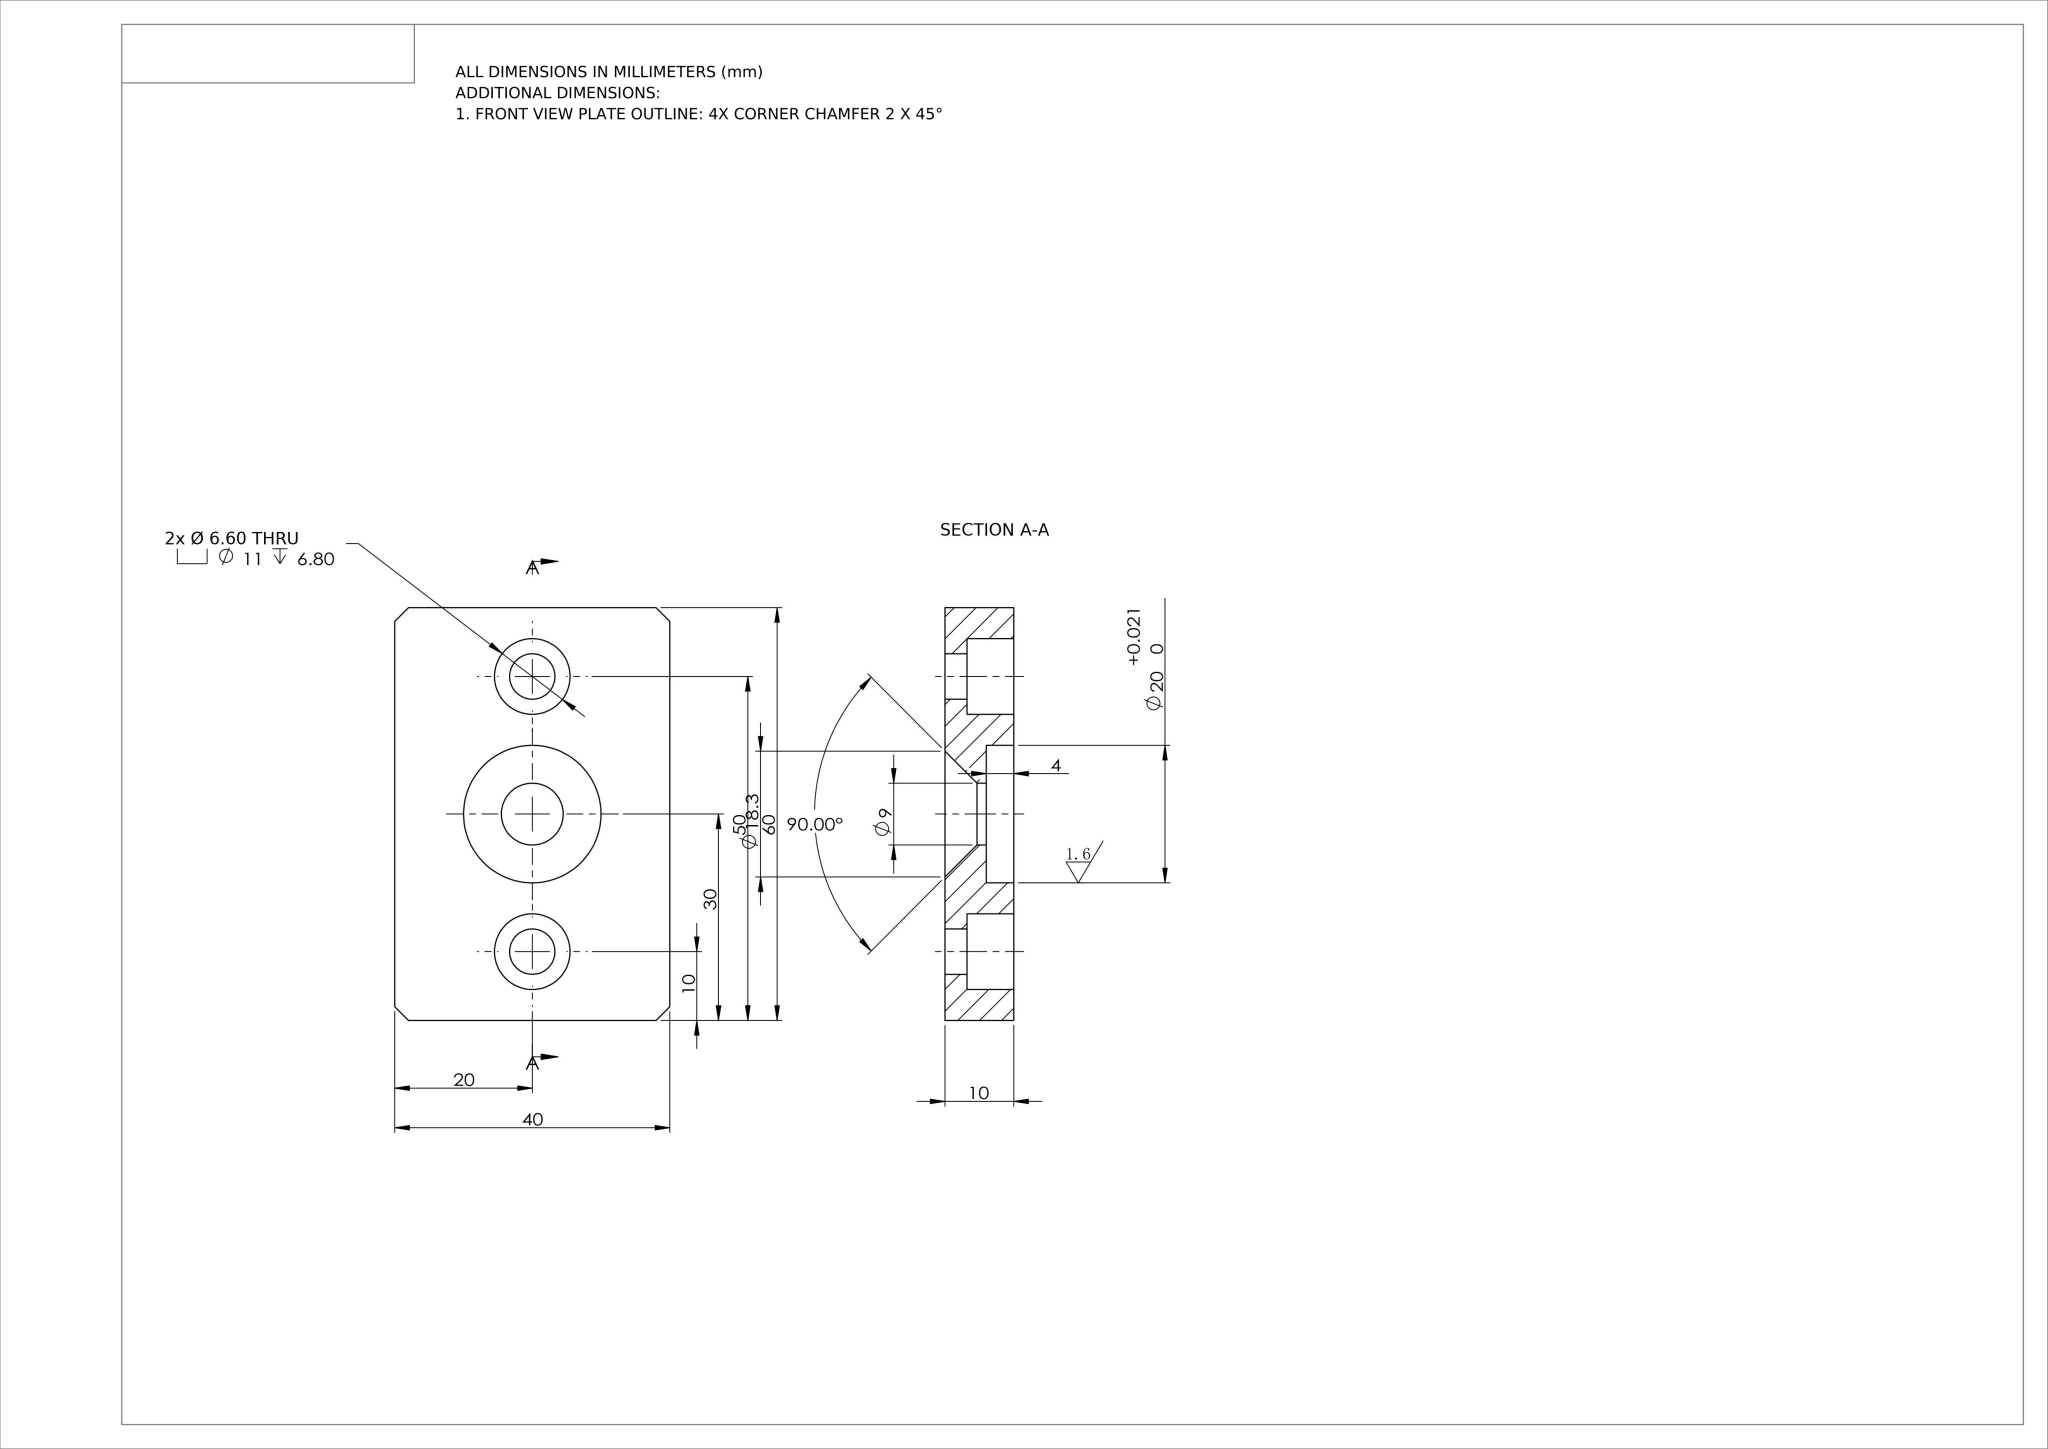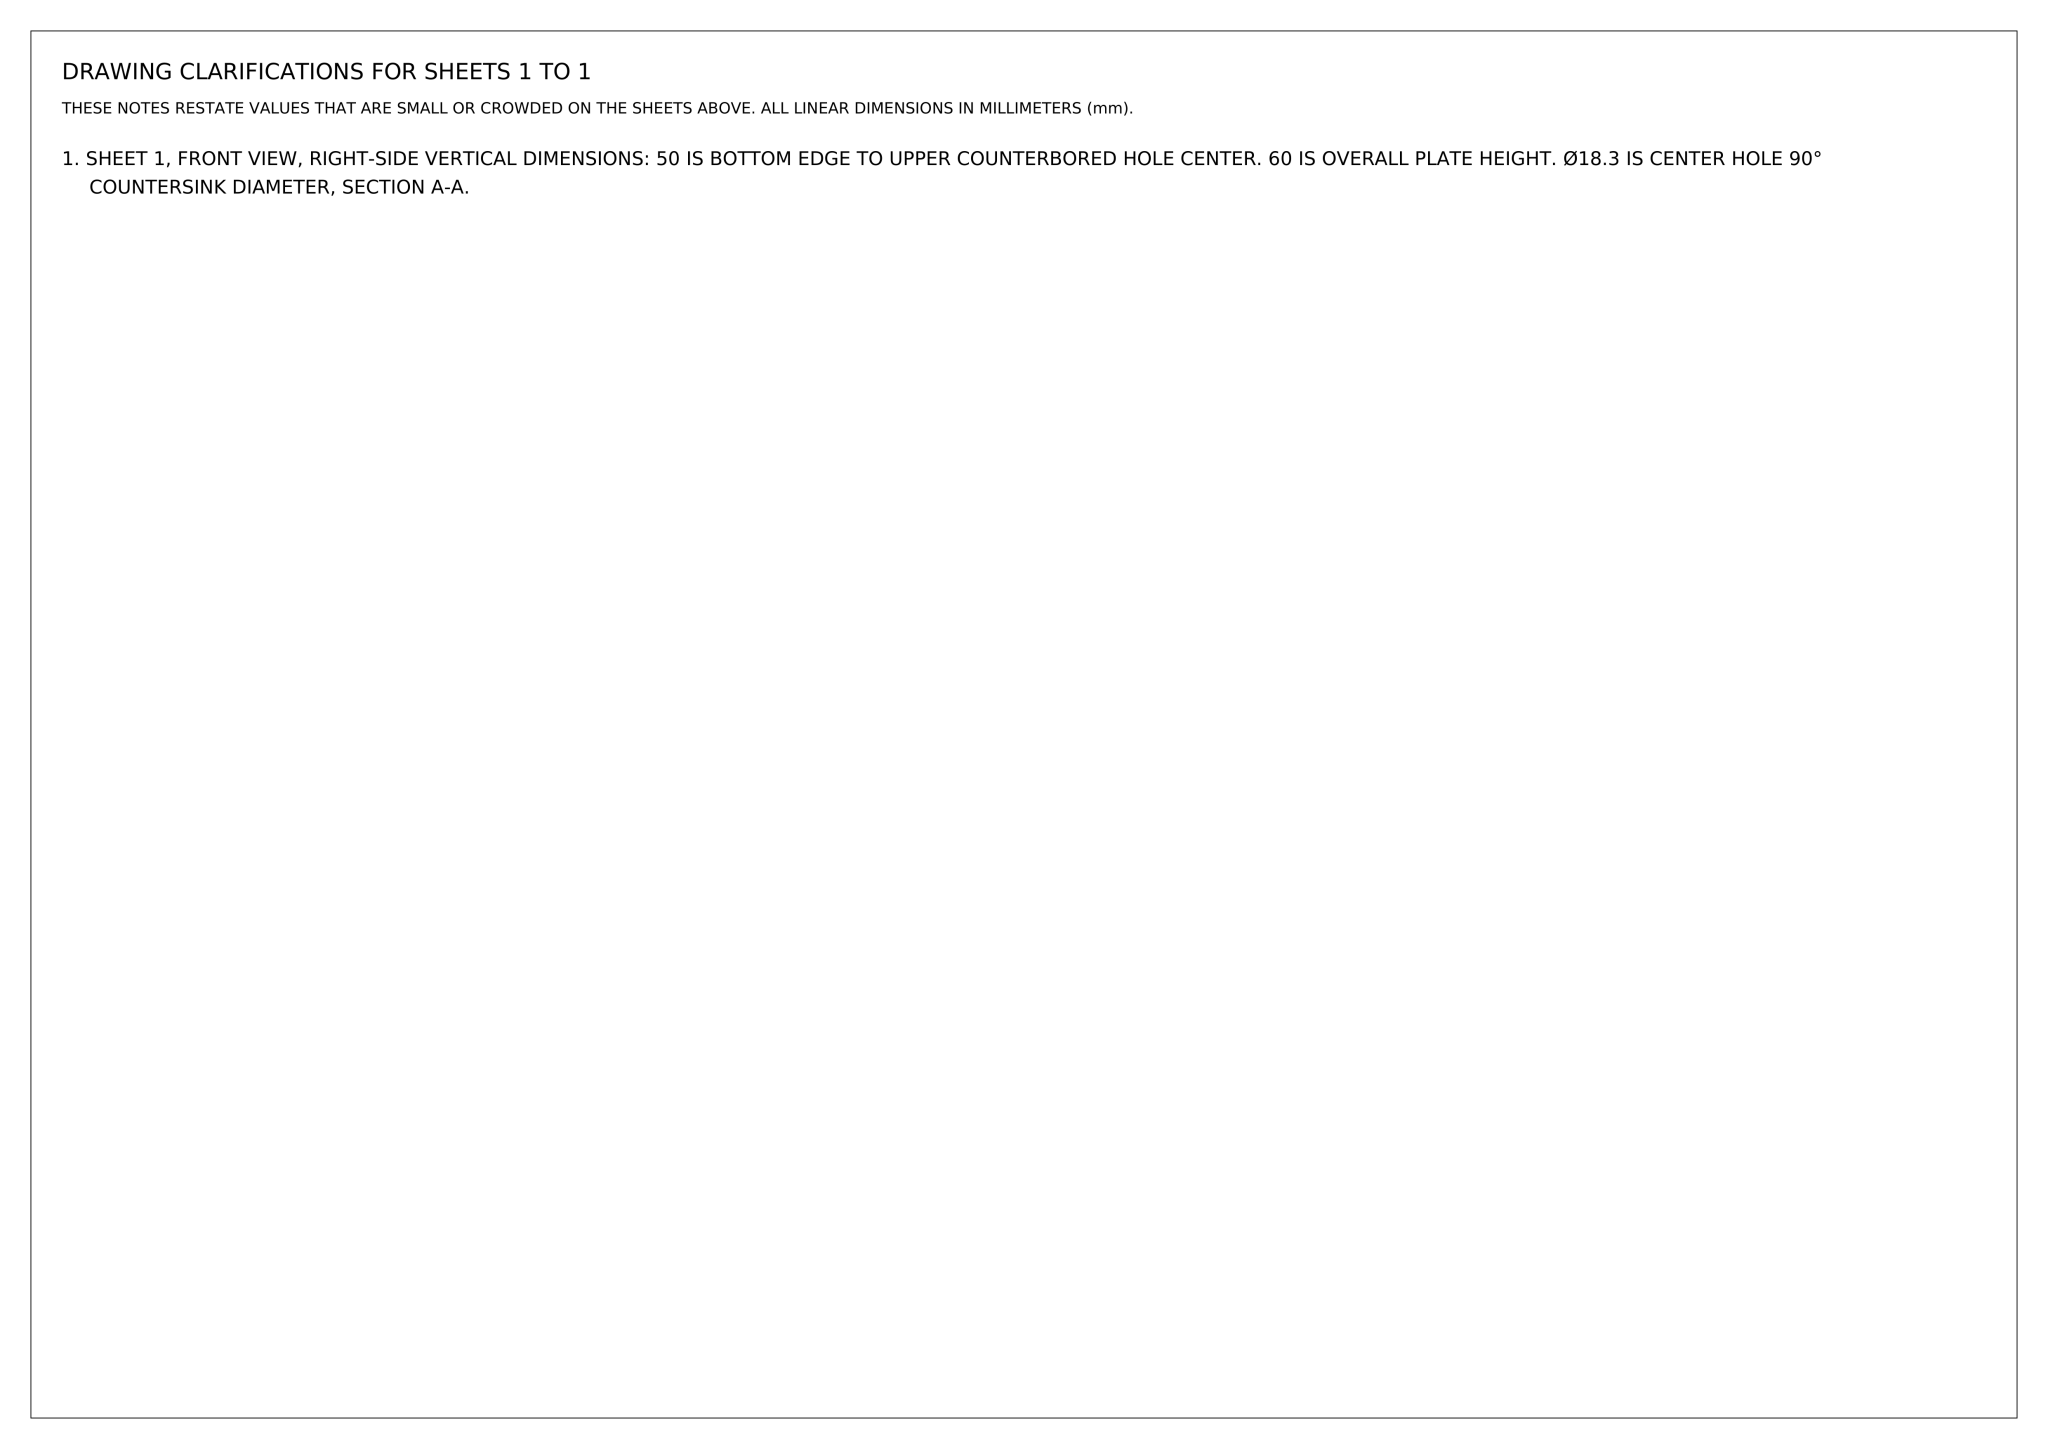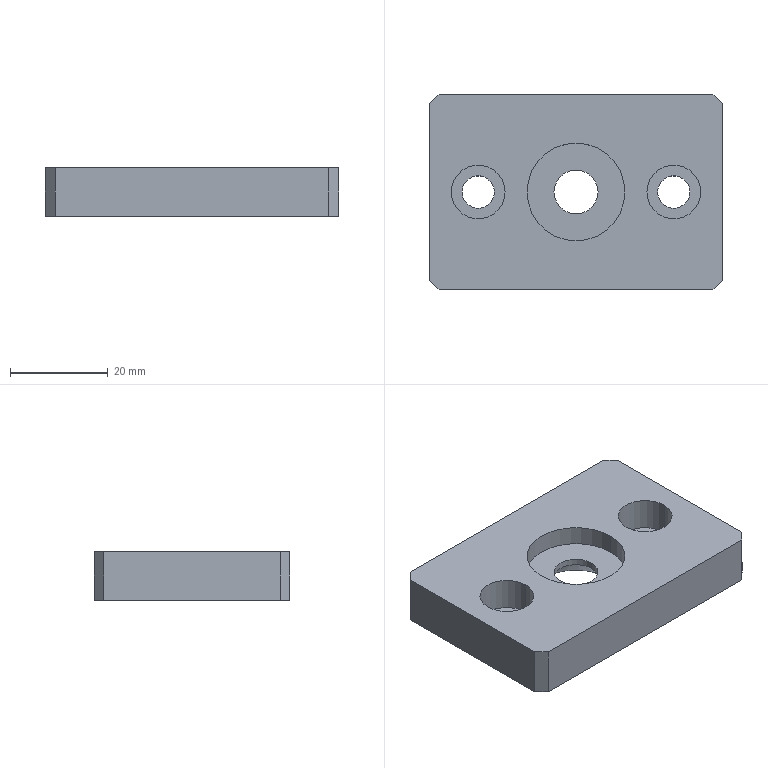Part | NX | mm | 1 solid | 27 faces | box 60 x 40 x 10 mm | volume 20359 mm3 | plane 13 | cylinder 12 | cone 2 | commonest cylinder face diameters 11 x4 6.6 x4 9 x2 20 x2
STEP:
#1=COLOUR_RGB('',0.6157,0.6431,0.6745);
#2=FILL_AREA_STYLE_COLOUR('',#1);
#3=FILL_AREA_STYLE('',(#2));
#4=SURFACE_STYLE_FILL_AREA(#3);
#5=SURFACE_SIDE_STYLE('',(#4));
#6=SURFACE_STYLE_USAGE(.BOTH.,#5);
#7=PRESENTATION_STYLE_ASSIGNMENT((#6));
#8=CARTESIAN_POINT('',(-25.5,-0.,3.2));
#9=VERTEX_POINT('',#8);
#10=CARTESIAN_POINT('',(-14.5,-0.,3.2));
#11=VERTEX_POINT('',#10);
#12=CARTESIAN_POINT('',(-20.,-0.,3.2));
#13=DIRECTION('',(0.,0.,1.));
#14=DIRECTION('',(1.,0.,0.));
#15=AXIS2_PLACEMENT_3D('',#12,#13,#14);
#16=CIRCLE('',#15,5.5);
#17=EDGE_CURVE('',#9,#11,#16,.T.);
#18=ORIENTED_EDGE('',*,*,#17,.F.);
#19=CARTESIAN_POINT('',(-25.5,-0.,10.));
#20=VERTEX_POINT('',#19);
#21=CARTESIAN_POINT('',(-25.5,-0.,10.));
#22=DIRECTION('',(0.,0.,1.));
#23=VECTOR('',#22,1000.);
#24=LINE('',#21,#23);
#25=EDGE_CURVE('',#9,#20,#24,.T.);
#26=ORIENTED_EDGE('',*,*,#25,.T.);
#27=CARTESIAN_POINT('',(-14.5,-0.,10.));
#28=VERTEX_POINT('',#27);
#29=CARTESIAN_POINT('',(-20.,-0.,10.));
#30=DIRECTION('',(0.,0.,1.));
#31=DIRECTION('',(1.,0.,0.));
#32=AXIS2_PLACEMENT_3D('',#29,#30,#31);
#33=CIRCLE('',#32,5.5);
#34=EDGE_CURVE('',#20,#28,#33,.T.);
#35=ORIENTED_EDGE('',*,*,#34,.T.);
#36=CARTESIAN_POINT('',(-14.5,-0.,10.));
#37=DIRECTION('',(0.,0.,1.));
#38=VECTOR('',#37,1000.);
#39=LINE('',#36,#38);
#40=EDGE_CURVE('',#11,#28,#39,.T.);
#41=ORIENTED_EDGE('',*,*,#40,.F.);
#42=EDGE_LOOP('',(#18,#26,#35,#41));
#43=FACE_OUTER_BOUND('',#42,.T.);
#44=CARTESIAN_POINT('',(-20.,-0.,10.));
#45=DIRECTION('',(0.,0.,1.));
#46=DIRECTION('',(1.,0.,0.));
#47=AXIS2_PLACEMENT_3D('',#44,#45,#46);
#48=CYLINDRICAL_SURFACE('',#47,5.5);
#49=ADVANCED_FACE('',(#43),#48,.F.);
#50=CARTESIAN_POINT('',(-23.3,-0.,0.));
#51=VERTEX_POINT('',#50);
#52=CARTESIAN_POINT('',(-16.7,-0.,0.));
#53=VERTEX_POINT('',#52);
#54=CARTESIAN_POINT('',(-20.,-0.,0.));
#55=DIRECTION('',(0.,0.,1.));
#56=DIRECTION('',(1.,0.,0.));
#57=AXIS2_PLACEMENT_3D('',#54,#55,#56);
#58=CIRCLE('',#57,3.3);
#59=EDGE_CURVE('',#51,#53,#58,.T.);
#60=ORIENTED_EDGE('',*,*,#59,.F.);
#61=CARTESIAN_POINT('',(-23.3,-0.,3.2));
#62=VERTEX_POINT('',#61);
#63=CARTESIAN_POINT('',(-23.3,-0.,10.));
#64=DIRECTION('',(0.,0.,1.));
#65=VECTOR('',#64,1000.);
#66=LINE('',#63,#65);
#67=EDGE_CURVE('',#51,#62,#66,.T.);
#68=ORIENTED_EDGE('',*,*,#67,.T.);
#69=CARTESIAN_POINT('',(-16.7,-0.,3.2));
#70=VERTEX_POINT('',#69);
#71=CARTESIAN_POINT('',(-20.,-0.,3.2));
#72=DIRECTION('',(0.,0.,1.));
#73=DIRECTION('',(1.,0.,0.));
#74=AXIS2_PLACEMENT_3D('',#71,#72,#73);
#75=CIRCLE('',#74,3.3);
#76=EDGE_CURVE('',#62,#70,#75,.T.);
#77=ORIENTED_EDGE('',*,*,#76,.T.);
#78=CARTESIAN_POINT('',(-16.7,-0.,10.));
#79=DIRECTION('',(0.,0.,1.));
#80=VECTOR('',#79,1000.);
#81=LINE('',#78,#80);
#82=EDGE_CURVE('',#53,#70,#81,.T.);
#83=ORIENTED_EDGE('',*,*,#82,.F.);
#84=EDGE_LOOP('',(#60,#68,#77,#83));
#85=FACE_OUTER_BOUND('',#84,.T.);
#86=CARTESIAN_POINT('',(-20.,-0.,10.));
#87=DIRECTION('',(0.,0.,1.));
#88=DIRECTION('',(1.,0.,0.));
#89=AXIS2_PLACEMENT_3D('',#86,#87,#88);
#90=CYLINDRICAL_SURFACE('',#89,3.3);
#91=ADVANCED_FACE('',(#85),#90,.F.);
#92=CARTESIAN_POINT('',(14.5,0.,3.2));
#93=VERTEX_POINT('',#92);
#94=CARTESIAN_POINT('',(25.5,0.,3.2));
#95=VERTEX_POINT('',#94);
#96=CARTESIAN_POINT('',(20.,0.,3.2));
#97=DIRECTION('',(0.,0.,1.));
#98=DIRECTION('',(1.,0.,0.));
#99=AXIS2_PLACEMENT_3D('',#96,#97,#98);
#100=CIRCLE('',#99,5.5);
#101=EDGE_CURVE('',#93,#95,#100,.T.);
#102=ORIENTED_EDGE('',*,*,#101,.F.);
#103=CARTESIAN_POINT('',(14.5,0.,10.));
#104=VERTEX_POINT('',#103);
#105=CARTESIAN_POINT('',(14.5,0.,10.));
#106=DIRECTION('',(0.,0.,1.));
#107=VECTOR('',#106,1000.);
#108=LINE('',#105,#107);
#109=EDGE_CURVE('',#93,#104,#108,.T.);
#110=ORIENTED_EDGE('',*,*,#109,.T.);
#111=CARTESIAN_POINT('',(25.5,0.,10.));
#112=VERTEX_POINT('',#111);
#113=CARTESIAN_POINT('',(20.,0.,10.));
#114=DIRECTION('',(0.,0.,1.));
#115=DIRECTION('',(1.,0.,0.));
#116=AXIS2_PLACEMENT_3D('',#113,#114,#115);
#117=CIRCLE('',#116,5.5);
#118=EDGE_CURVE('',#104,#112,#117,.T.);
#119=ORIENTED_EDGE('',*,*,#118,.T.);
#120=CARTESIAN_POINT('',(25.5,0.,10.));
#121=DIRECTION('',(0.,0.,1.));
#122=VECTOR('',#121,1000.);
#123=LINE('',#120,#122);
#124=EDGE_CURVE('',#95,#112,#123,.T.);
#125=ORIENTED_EDGE('',*,*,#124,.F.);
#126=EDGE_LOOP('',(#102,#110,#119,#125));
#127=FACE_OUTER_BOUND('',#126,.T.);
#128=CARTESIAN_POINT('',(20.,0.,10.));
#129=DIRECTION('',(0.,0.,1.));
#130=DIRECTION('',(1.,0.,0.));
#131=AXIS2_PLACEMENT_3D('',#128,#129,#130);
#132=CYLINDRICAL_SURFACE('',#131,5.5);
#133=ADVANCED_FACE('',(#127),#132,.F.);
#134=CARTESIAN_POINT('',(16.7,0.,0.));
#135=VERTEX_POINT('',#134);
#136=CARTESIAN_POINT('',(23.3,0.,0.));
#137=VERTEX_POINT('',#136);
#138=CARTESIAN_POINT('',(20.,0.,0.));
#139=DIRECTION('',(0.,0.,1.));
#140=DIRECTION('',(1.,0.,0.));
#141=AXIS2_PLACEMENT_3D('',#138,#139,#140);
#142=CIRCLE('',#141,3.3);
#143=EDGE_CURVE('',#135,#137,#142,.T.);
#144=ORIENTED_EDGE('',*,*,#143,.F.);
#145=CARTESIAN_POINT('',(16.7,0.,3.2));
#146=VERTEX_POINT('',#145);
#147=CARTESIAN_POINT('',(16.7,0.,10.));
#148=DIRECTION('',(0.,0.,1.));
#149=VECTOR('',#148,1000.);
#150=LINE('',#147,#149);
#151=EDGE_CURVE('',#135,#146,#150,.T.);
#152=ORIENTED_EDGE('',*,*,#151,.T.);
#153=CARTESIAN_POINT('',(23.3,0.,3.2));
#154=VERTEX_POINT('',#153);
#155=CARTESIAN_POINT('',(20.,0.,3.2));
#156=DIRECTION('',(0.,0.,1.));
#157=DIRECTION('',(1.,0.,0.));
#158=AXIS2_PLACEMENT_3D('',#155,#156,#157);
#159=CIRCLE('',#158,3.3);
#160=EDGE_CURVE('',#146,#154,#159,.T.);
#161=ORIENTED_EDGE('',*,*,#160,.T.);
#162=CARTESIAN_POINT('',(23.3,0.,10.));
#163=DIRECTION('',(0.,0.,1.));
#164=VECTOR('',#163,1000.);
#165=LINE('',#162,#164);
#166=EDGE_CURVE('',#137,#154,#165,.T.);
#167=ORIENTED_EDGE('',*,*,#166,.F.);
#168=EDGE_LOOP('',(#144,#152,#161,#167));
#169=FACE_OUTER_BOUND('',#168,.T.);
#170=CARTESIAN_POINT('',(20.,0.,10.));
#171=DIRECTION('',(0.,0.,1.));
#172=DIRECTION('',(1.,0.,0.));
#173=AXIS2_PLACEMENT_3D('',#170,#171,#172);
#174=CYLINDRICAL_SURFACE('',#173,3.3);
#175=ADVANCED_FACE('',(#169),#174,.F.);
#176=CARTESIAN_POINT('',(4.5,0.,4.65));
#177=VERTEX_POINT('',#176);
#178=CARTESIAN_POINT('',(-4.5,-0.,4.65));
#179=VERTEX_POINT('',#178);
#180=CARTESIAN_POINT('',(0.,0.,4.65));
#181=DIRECTION('',(-0.,-0.,-1.));
#182=DIRECTION('',(-1.,-0.,-0.));
#183=AXIS2_PLACEMENT_3D('',#180,#181,#182);
#184=CIRCLE('',#183,4.5);
#185=EDGE_CURVE('',#177,#179,#184,.T.);
#186=ORIENTED_EDGE('',*,*,#185,.F.);
#187=CARTESIAN_POINT('',(9.15,0.,-0.));
#188=VERTEX_POINT('',#187);
#189=CARTESIAN_POINT('',(9.15,0.,0.));
#190=DIRECTION('',(0.7071,0.,-0.7071));
#191=VECTOR('',#190,1000.);
#192=LINE('',#189,#191);
#193=EDGE_CURVE('',#177,#188,#192,.T.);
#194=ORIENTED_EDGE('',*,*,#193,.T.);
#195=CARTESIAN_POINT('',(-9.15,-0.,0.));
#196=VERTEX_POINT('',#195);
#197=CARTESIAN_POINT('',(0.,0.,0.));
#198=DIRECTION('',(-0.,-0.,-1.));
#199=DIRECTION('',(-1.,-0.,-0.));
#200=AXIS2_PLACEMENT_3D('',#197,#198,#199);
#201=CIRCLE('',#200,9.15);
#202=EDGE_CURVE('',#188,#196,#201,.T.);
#203=ORIENTED_EDGE('',*,*,#202,.T.);
#204=CARTESIAN_POINT('',(-9.15,-0.,-0.));
#205=DIRECTION('',(-0.7071,-0.,-0.7071));
#206=VECTOR('',#205,1000.);
#207=LINE('',#204,#206);
#208=EDGE_CURVE('',#179,#196,#207,.T.);
#209=ORIENTED_EDGE('',*,*,#208,.F.);
#210=EDGE_LOOP('',(#186,#194,#203,#209));
#211=FACE_OUTER_BOUND('',#210,.T.);
#212=CARTESIAN_POINT('',(0.,0.,0.));
#213=DIRECTION('',(-0.,-0.,-1.));
#214=DIRECTION('',(-1.,-0.,-0.));
#215=AXIS2_PLACEMENT_3D('',#212,#213,#214);
#216=CONICAL_SURFACE('',#215,9.15,0.7854);
#217=ADVANCED_FACE('',(#211),#216,.F.);
#218=CARTESIAN_POINT('',(-4.5,-0.,6.));
#219=VERTEX_POINT('',#218);
#220=CARTESIAN_POINT('',(4.5,0.,6.));
#221=VERTEX_POINT('',#220);
#222=CARTESIAN_POINT('',(0.,0.,6.));
#223=DIRECTION('',(0.,0.,1.));
#224=DIRECTION('',(1.,0.,0.));
#225=AXIS2_PLACEMENT_3D('',#222,#223,#224);
#226=CIRCLE('',#225,4.5);
#227=EDGE_CURVE('',#219,#221,#226,.T.);
#228=ORIENTED_EDGE('',*,*,#227,.T.);
#229=CARTESIAN_POINT('',(4.5,0.,0.));
#230=DIRECTION('',(-0.,-0.,-1.));
#231=VECTOR('',#230,1000.);
#232=LINE('',#229,#231);
#233=EDGE_CURVE('',#221,#177,#232,.T.);
#234=ORIENTED_EDGE('',*,*,#233,.T.);
#235=ORIENTED_EDGE('',*,*,#185,.T.);
#236=CARTESIAN_POINT('',(-4.5,-0.,-0.));
#237=DIRECTION('',(-0.,-0.,-1.));
#238=VECTOR('',#237,1000.);
#239=LINE('',#236,#238);
#240=EDGE_CURVE('',#219,#179,#239,.T.);
#241=ORIENTED_EDGE('',*,*,#240,.F.);
#242=EDGE_LOOP('',(#228,#234,#235,#241));
#243=FACE_OUTER_BOUND('',#242,.T.);
#244=CARTESIAN_POINT('',(0.,0.,0.));
#245=DIRECTION('',(-0.,-0.,-1.));
#246=DIRECTION('',(-1.,-0.,-0.));
#247=AXIS2_PLACEMENT_3D('',#244,#245,#246);
#248=CYLINDRICAL_SURFACE('',#247,4.5);
#249=ADVANCED_FACE('',(#243),#248,.F.);
#250=CARTESIAN_POINT('',(-10.,-0.,6.));
#251=VERTEX_POINT('',#250);
#252=CARTESIAN_POINT('',(10.,0.,6.));
#253=VERTEX_POINT('',#252);
#254=CARTESIAN_POINT('',(0.,0.,6.));
#255=DIRECTION('',(0.,0.,1.));
#256=DIRECTION('',(1.,0.,0.));
#257=AXIS2_PLACEMENT_3D('',#254,#255,#256);
#258=CIRCLE('',#257,10.);
#259=EDGE_CURVE('',#251,#253,#258,.T.);
#260=ORIENTED_EDGE('',*,*,#259,.F.);
#261=CARTESIAN_POINT('',(-10.,-0.,10.));
#262=VERTEX_POINT('',#261);
#263=CARTESIAN_POINT('',(-10.,-0.,6.));
#264=DIRECTION('',(0.,0.,1.));
#265=VECTOR('',#264,1000.);
#266=LINE('',#263,#265);
#267=EDGE_CURVE('',#251,#262,#266,.T.);
#268=ORIENTED_EDGE('',*,*,#267,.T.);
#269=CARTESIAN_POINT('',(10.,0.,10.));
#270=VERTEX_POINT('',#269);
#271=CARTESIAN_POINT('',(0.,0.,10.));
#272=DIRECTION('',(0.,0.,1.));
#273=DIRECTION('',(1.,0.,0.));
#274=AXIS2_PLACEMENT_3D('',#271,#272,#273);
#275=CIRCLE('',#274,10.);
#276=EDGE_CURVE('',#262,#270,#275,.T.);
#277=ORIENTED_EDGE('',*,*,#276,.T.);
#278=CARTESIAN_POINT('',(10.,0.,6.));
#279=DIRECTION('',(0.,0.,1.));
#280=VECTOR('',#279,1000.);
#281=LINE('',#278,#280);
#282=EDGE_CURVE('',#253,#270,#281,.T.);
#283=ORIENTED_EDGE('',*,*,#282,.F.);
#284=EDGE_LOOP('',(#260,#268,#277,#283));
#285=FACE_OUTER_BOUND('',#284,.T.);
#286=CARTESIAN_POINT('',(0.,0.,6.));
#287=DIRECTION('',(0.,0.,1.));
#288=DIRECTION('',(1.,0.,0.));
#289=AXIS2_PLACEMENT_3D('',#286,#287,#288);
#290=CYLINDRICAL_SURFACE('',#289,10.);
#291=ADVANCED_FACE('',(#285),#290,.F.);
#292=CARTESIAN_POINT('',(30.,-18.,10.));
#293=VERTEX_POINT('',#292);
#294=CARTESIAN_POINT('',(30.,18.,10.));
#295=VERTEX_POINT('',#294);
#296=CARTESIAN_POINT('',(30.,-20.,10.));
#297=DIRECTION('',(0.,1.,0.));
#298=VECTOR('',#297,1000.);
#299=LINE('',#296,#298);
#300=EDGE_CURVE('',#293,#295,#299,.T.);
#301=ORIENTED_EDGE('',*,*,#300,.F.);
#302=CARTESIAN_POINT('',(30.,-18.,0.));
#303=VERTEX_POINT('',#302);
#304=CARTESIAN_POINT('',(30.,-18.,10.));
#305=DIRECTION('',(-0.,-0.,-1.));
#306=VECTOR('',#305,1000.);
#307=LINE('',#304,#306);
#308=EDGE_CURVE('',#293,#303,#307,.T.);
#309=ORIENTED_EDGE('',*,*,#308,.T.);
#310=CARTESIAN_POINT('',(30.,18.,0.));
#311=VERTEX_POINT('',#310);
#312=CARTESIAN_POINT('',(30.,-20.,0.));
#313=DIRECTION('',(0.,1.,0.));
#314=VECTOR('',#313,1000.);
#315=LINE('',#312,#314);
#316=EDGE_CURVE('',#303,#311,#315,.T.);
#317=ORIENTED_EDGE('',*,*,#316,.T.);
#318=CARTESIAN_POINT('',(30.,18.,10.));
#319=DIRECTION('',(0.,0.,1.));
#320=VECTOR('',#319,1000.);
#321=LINE('',#318,#320);
#322=EDGE_CURVE('',#311,#295,#321,.T.);
#323=ORIENTED_EDGE('',*,*,#322,.T.);
#324=EDGE_LOOP('',(#301,#309,#317,#323));
#325=FACE_OUTER_BOUND('',#324,.T.);
#326=CARTESIAN_POINT('',(30.,-20.,10.));
#327=DIRECTION('',(-1.,-0.,0.));
#328=DIRECTION('',(0.,0.,1.));
#329=AXIS2_PLACEMENT_3D('',#326,#327,#328);
#330=PLANE('',#329);
#331=ADVANCED_FACE('',(#325),#330,.F.);
#332=CARTESIAN_POINT('',(28.,20.,0.));
#333=VERTEX_POINT('',#332);
#334=CARTESIAN_POINT('',(-28.,20.,0.));
#335=VERTEX_POINT('',#334);
#336=CARTESIAN_POINT('',(-30.,20.,0.));
#337=DIRECTION('',(-1.,-0.,-0.));
#338=VECTOR('',#337,1000.);
#339=LINE('',#336,#338);
#340=EDGE_CURVE('',#333,#335,#339,.T.);
#341=ORIENTED_EDGE('',*,*,#340,.T.);
#342=CARTESIAN_POINT('',(-28.,20.,10.));
#343=VERTEX_POINT('',#342);
#344=CARTESIAN_POINT('',(-28.,20.,10.));
#345=DIRECTION('',(0.,0.,1.));
#346=VECTOR('',#345,1000.);
#347=LINE('',#344,#346);
#348=EDGE_CURVE('',#335,#343,#347,.T.);
#349=ORIENTED_EDGE('',*,*,#348,.T.);
#350=CARTESIAN_POINT('',(28.,20.,10.));
#351=VERTEX_POINT('',#350);
#352=CARTESIAN_POINT('',(-30.,20.,10.));
#353=DIRECTION('',(-1.,-0.,-0.));
#354=VECTOR('',#353,1000.);
#355=LINE('',#352,#354);
#356=EDGE_CURVE('',#351,#343,#355,.T.);
#357=ORIENTED_EDGE('',*,*,#356,.F.);
#358=CARTESIAN_POINT('',(28.,20.,10.));
#359=DIRECTION('',(-0.,-0.,-1.));
#360=VECTOR('',#359,1000.);
#361=LINE('',#358,#360);
#362=EDGE_CURVE('',#351,#333,#361,.T.);
#363=ORIENTED_EDGE('',*,*,#362,.T.);
#364=EDGE_LOOP('',(#341,#349,#357,#363));
#365=FACE_OUTER_BOUND('',#364,.T.);
#366=CARTESIAN_POINT('',(-30.,20.,10.));
#367=DIRECTION('',(-0.,-1.,0.));
#368=DIRECTION('',(-0.,-0.,-1.));
#369=AXIS2_PLACEMENT_3D('',#366,#367,#368);
#370=PLANE('',#369);
#371=ADVANCED_FACE('',(#365),#370,.F.);
#372=CARTESIAN_POINT('',(-30.,18.,0.));
#373=VERTEX_POINT('',#372);
#374=CARTESIAN_POINT('',(-30.,-18.,0.));
#375=VERTEX_POINT('',#374);
#376=CARTESIAN_POINT('',(-30.,-20.,0.));
#377=DIRECTION('',(-0.,-1.,-0.));
#378=VECTOR('',#377,1000.);
#379=LINE('',#376,#378);
#380=EDGE_CURVE('',#373,#375,#379,.T.);
#381=ORIENTED_EDGE('',*,*,#380,.T.);
#382=CARTESIAN_POINT('',(-30.,-18.,10.));
#383=VERTEX_POINT('',#382);
#384=CARTESIAN_POINT('',(-30.,-18.,10.));
#385=DIRECTION('',(0.,0.,1.));
#386=VECTOR('',#385,1000.);
#387=LINE('',#384,#386);
#388=EDGE_CURVE('',#375,#383,#387,.T.);
#389=ORIENTED_EDGE('',*,*,#388,.T.);
#390=CARTESIAN_POINT('',(-30.,18.,10.));
#391=VERTEX_POINT('',#390);
#392=CARTESIAN_POINT('',(-30.,-20.,10.));
#393=DIRECTION('',(-0.,-1.,-0.));
#394=VECTOR('',#393,1000.);
#395=LINE('',#392,#394);
#396=EDGE_CURVE('',#391,#383,#395,.T.);
#397=ORIENTED_EDGE('',*,*,#396,.F.);
#398=CARTESIAN_POINT('',(-30.,18.,10.));
#399=DIRECTION('',(-0.,-0.,-1.));
#400=VECTOR('',#399,1000.);
#401=LINE('',#398,#400);
#402=EDGE_CURVE('',#391,#373,#401,.T.);
#403=ORIENTED_EDGE('',*,*,#402,.T.);
#404=EDGE_LOOP('',(#381,#389,#397,#403));
#405=FACE_OUTER_BOUND('',#404,.T.);
#406=CARTESIAN_POINT('',(-30.,-20.,10.));
#407=DIRECTION('',(1.,0.,-0.));
#408=DIRECTION('',(-0.,-0.,-1.));
#409=AXIS2_PLACEMENT_3D('',#406,#407,#408);
#410=PLANE('',#409);
#411=ADVANCED_FACE('',(#405),#410,.F.);
#412=CARTESIAN_POINT('',(-28.,-20.,10.));
#413=VERTEX_POINT('',#412);
#414=CARTESIAN_POINT('',(28.,-20.,10.));
#415=VERTEX_POINT('',#414);
#416=CARTESIAN_POINT('',(-30.,-20.,10.));
#417=DIRECTION('',(1.,0.,0.));
#418=VECTOR('',#417,1000.);
#419=LINE('',#416,#418);
#420=EDGE_CURVE('',#413,#415,#419,.T.);
#421=ORIENTED_EDGE('',*,*,#420,.F.);
#422=CARTESIAN_POINT('',(-28.,-20.,0.));
#423=VERTEX_POINT('',#422);
#424=CARTESIAN_POINT('',(-28.,-20.,10.));
#425=DIRECTION('',(-0.,-0.,-1.));
#426=VECTOR('',#425,1000.);
#427=LINE('',#424,#426);
#428=EDGE_CURVE('',#413,#423,#427,.T.);
#429=ORIENTED_EDGE('',*,*,#428,.T.);
#430=CARTESIAN_POINT('',(28.,-20.,0.));
#431=VERTEX_POINT('',#430);
#432=CARTESIAN_POINT('',(-30.,-20.,0.));
#433=DIRECTION('',(1.,0.,0.));
#434=VECTOR('',#433,1000.);
#435=LINE('',#432,#434);
#436=EDGE_CURVE('',#423,#431,#435,.T.);
#437=ORIENTED_EDGE('',*,*,#436,.T.);
#438=CARTESIAN_POINT('',(28.,-20.,10.));
#439=DIRECTION('',(0.,0.,1.));
#440=VECTOR('',#439,1000.);
#441=LINE('',#438,#440);
#442=EDGE_CURVE('',#431,#415,#441,.T.);
#443=ORIENTED_EDGE('',*,*,#442,.T.);
#444=EDGE_LOOP('',(#421,#429,#437,#443));
#445=FACE_OUTER_BOUND('',#444,.T.);
#446=CARTESIAN_POINT('',(-30.,-20.,10.));
#447=DIRECTION('',(0.,1.,-0.));
#448=DIRECTION('',(0.,0.,1.));
#449=AXIS2_PLACEMENT_3D('',#446,#447,#448);
#450=PLANE('',#449);
#451=ADVANCED_FACE('',(#445),#450,.F.);
#452=CARTESIAN_POINT('',(-20.,-0.,10.));
#453=DIRECTION('',(0.,0.,1.));
#454=DIRECTION('',(1.,0.,0.));
#455=AXIS2_PLACEMENT_3D('',#452,#453,#454);
#456=CIRCLE('',#455,5.5);
#457=EDGE_CURVE('',#28,#20,#456,.T.);
#458=ORIENTED_EDGE('',*,*,#457,.F.);
#459=ORIENTED_EDGE('',*,*,#34,.F.);
#460=EDGE_LOOP('',(#458,#459));
#461=FACE_BOUND('',#460,.T.);
#462=CARTESIAN_POINT('',(20.,0.,10.));
#463=DIRECTION('',(0.,0.,1.));
#464=DIRECTION('',(1.,0.,0.));
#465=AXIS2_PLACEMENT_3D('',#462,#463,#464);
#466=CIRCLE('',#465,5.5);
#467=EDGE_CURVE('',#112,#104,#466,.T.);
#468=ORIENTED_EDGE('',*,*,#467,.F.);
#469=ORIENTED_EDGE('',*,*,#118,.F.);
#470=EDGE_LOOP('',(#468,#469));
#471=FACE_BOUND('',#470,.T.);
#472=CARTESIAN_POINT('',(0.,0.,10.));
#473=DIRECTION('',(0.,0.,1.));
#474=DIRECTION('',(1.,0.,0.));
#475=AXIS2_PLACEMENT_3D('',#472,#473,#474);
#476=CIRCLE('',#475,10.);
#477=EDGE_CURVE('',#270,#262,#476,.T.);
#478=ORIENTED_EDGE('',*,*,#477,.F.);
#479=ORIENTED_EDGE('',*,*,#276,.F.);
#480=EDGE_LOOP('',(#478,#479));
#481=FACE_BOUND('',#480,.T.);
#482=ORIENTED_EDGE('',*,*,#396,.T.);
#483=CARTESIAN_POINT('',(-28.,-20.,10.));
#484=DIRECTION('',(0.7071,-0.7071,0.));
#485=VECTOR('',#484,1000.);
#486=LINE('',#483,#485);
#487=EDGE_CURVE('',#383,#413,#486,.T.);
#488=ORIENTED_EDGE('',*,*,#487,.T.);
#489=ORIENTED_EDGE('',*,*,#420,.T.);
#490=CARTESIAN_POINT('',(30.,-18.,10.));
#491=DIRECTION('',(0.7071,0.7071,0.));
#492=VECTOR('',#491,1000.);
#493=LINE('',#490,#492);
#494=EDGE_CURVE('',#415,#293,#493,.T.);
#495=ORIENTED_EDGE('',*,*,#494,.T.);
#496=ORIENTED_EDGE('',*,*,#300,.T.);
#497=CARTESIAN_POINT('',(28.,20.,10.));
#498=DIRECTION('',(-0.7071,0.7071,-0.));
#499=VECTOR('',#498,1000.);
#500=LINE('',#497,#499);
#501=EDGE_CURVE('',#295,#351,#500,.T.);
#502=ORIENTED_EDGE('',*,*,#501,.T.);
#503=ORIENTED_EDGE('',*,*,#356,.T.);
#504=CARTESIAN_POINT('',(-30.,18.,10.));
#505=DIRECTION('',(-0.7071,-0.7071,-0.));
#506=VECTOR('',#505,1000.);
#507=LINE('',#504,#506);
#508=EDGE_CURVE('',#343,#391,#507,.T.);
#509=ORIENTED_EDGE('',*,*,#508,.T.);
#510=EDGE_LOOP('',(#482,#488,#489,#495,#496,#502,#503,#509));
#511=FACE_OUTER_BOUND('',#510,.T.);
#512=CARTESIAN_POINT('',(30.,20.,10.));
#513=DIRECTION('',(0.,-0.,-1.));
#514=DIRECTION('',(-1.,-0.,-0.));
#515=AXIS2_PLACEMENT_3D('',#512,#513,#514);
#516=PLANE('',#515);
#517=ADVANCED_FACE('',(#461,#471,#481,#511),#516,.F.);
#518=CARTESIAN_POINT('',(-20.,-0.,0.));
#519=DIRECTION('',(0.,0.,1.));
#520=DIRECTION('',(1.,0.,0.));
#521=AXIS2_PLACEMENT_3D('',#518,#519,#520);
#522=CIRCLE('',#521,3.3);
#523=EDGE_CURVE('',#53,#51,#522,.T.);
#524=ORIENTED_EDGE('',*,*,#523,.T.);
#525=ORIENTED_EDGE('',*,*,#59,.T.);
#526=EDGE_LOOP('',(#524,#525));
#527=FACE_BOUND('',#526,.T.);
#528=CARTESIAN_POINT('',(20.,0.,0.));
#529=DIRECTION('',(0.,0.,1.));
#530=DIRECTION('',(1.,0.,0.));
#531=AXIS2_PLACEMENT_3D('',#528,#529,#530);
#532=CIRCLE('',#531,3.3);
#533=EDGE_CURVE('',#137,#135,#532,.T.);
#534=ORIENTED_EDGE('',*,*,#533,.T.);
#535=ORIENTED_EDGE('',*,*,#143,.T.);
#536=EDGE_LOOP('',(#534,#535));
#537=FACE_BOUND('',#536,.T.);
#538=CARTESIAN_POINT('',(0.,0.,0.));
#539=DIRECTION('',(-0.,-0.,-1.));
#540=DIRECTION('',(-1.,-0.,-0.));
#541=AXIS2_PLACEMENT_3D('',#538,#539,#540);
#542=CIRCLE('',#541,9.15);
#543=EDGE_CURVE('',#196,#188,#542,.T.);
#544=ORIENTED_EDGE('',*,*,#543,.F.);
#545=ORIENTED_EDGE('',*,*,#202,.F.);
#546=EDGE_LOOP('',(#544,#545));
#547=FACE_BOUND('',#546,.T.);
#548=ORIENTED_EDGE('',*,*,#436,.F.);
#549=CARTESIAN_POINT('',(-19.,-29.,0.));
#550=DIRECTION('',(-0.7071,0.7071,-0.));
#551=VECTOR('',#550,1000.);
#552=LINE('',#549,#551);
#553=EDGE_CURVE('',#423,#375,#552,.T.);
#554=ORIENTED_EDGE('',*,*,#553,.T.);
#555=ORIENTED_EDGE('',*,*,#380,.F.);
#556=CARTESIAN_POINT('',(1.,49.,0.));
#557=DIRECTION('',(0.7071,0.7071,0.));
#558=VECTOR('',#557,1000.);
#559=LINE('',#556,#558);
#560=EDGE_CURVE('',#373,#335,#559,.T.);
#561=ORIENTED_EDGE('',*,*,#560,.T.);
#562=ORIENTED_EDGE('',*,*,#340,.F.);
#563=CARTESIAN_POINT('',(29.,19.,0.));
#564=DIRECTION('',(0.7071,-0.7071,0.));
#565=VECTOR('',#564,1000.);
#566=LINE('',#563,#565);
#567=EDGE_CURVE('',#333,#311,#566,.T.);
#568=ORIENTED_EDGE('',*,*,#567,.T.);
#569=ORIENTED_EDGE('',*,*,#316,.F.);
#570=CARTESIAN_POINT('',(49.,1.,0.));
#571=DIRECTION('',(-0.7071,-0.7071,-0.));
#572=VECTOR('',#571,1000.);
#573=LINE('',#570,#572);
#574=EDGE_CURVE('',#303,#431,#573,.T.);
#575=ORIENTED_EDGE('',*,*,#574,.T.);
#576=EDGE_LOOP('',(#548,#554,#555,#561,#562,#568,#569,#575));
#577=FACE_OUTER_BOUND('',#576,.T.);
#578=CARTESIAN_POINT('',(30.,20.,0.));
#579=DIRECTION('',(0.,-0.,-1.));
#580=DIRECTION('',(-1.,-0.,-0.));
#581=AXIS2_PLACEMENT_3D('',#578,#579,#580);
#582=PLANE('',#581);
#583=ADVANCED_FACE('',(#527,#537,#547,#577),#582,.T.);
#584=ORIENTED_EDGE('',*,*,#267,.F.);
#585=CARTESIAN_POINT('',(0.,0.,6.));
#586=DIRECTION('',(0.,0.,1.));
#587=DIRECTION('',(1.,0.,0.));
#588=AXIS2_PLACEMENT_3D('',#585,#586,#587);
#589=CIRCLE('',#588,10.);
#590=EDGE_CURVE('',#253,#251,#589,.T.);
#591=ORIENTED_EDGE('',*,*,#590,.F.);
#592=ORIENTED_EDGE('',*,*,#282,.T.);
#593=ORIENTED_EDGE('',*,*,#477,.T.);
#594=EDGE_LOOP('',(#584,#591,#592,#593));
#595=FACE_OUTER_BOUND('',#594,.T.);
#596=CARTESIAN_POINT('',(0.,0.,6.));
#597=DIRECTION('',(0.,0.,1.));
#598=DIRECTION('',(1.,0.,0.));
#599=AXIS2_PLACEMENT_3D('',#596,#597,#598);
#600=CYLINDRICAL_SURFACE('',#599,10.);
#601=ADVANCED_FACE('',(#595),#600,.F.);
#602=ORIENTED_EDGE('',*,*,#227,.F.);
#603=CARTESIAN_POINT('',(0.,0.,6.));
#604=DIRECTION('',(0.,0.,1.));
#605=DIRECTION('',(1.,0.,0.));
#606=AXIS2_PLACEMENT_3D('',#603,#604,#605);
#607=CIRCLE('',#606,4.5);
#608=EDGE_CURVE('',#221,#219,#607,.T.);
#609=ORIENTED_EDGE('',*,*,#608,.F.);
#610=EDGE_LOOP('',(#602,#609));
#611=FACE_BOUND('',#610,.T.);
#612=ORIENTED_EDGE('',*,*,#590,.T.);
#613=ORIENTED_EDGE('',*,*,#259,.T.);
#614=EDGE_LOOP('',(#612,#613));
#615=FACE_OUTER_BOUND('',#614,.T.);
#616=CARTESIAN_POINT('',(0.,0.,6.));
#617=DIRECTION('',(-0.,0.,1.));
#618=DIRECTION('',(1.,0.,0.));
#619=AXIS2_PLACEMENT_3D('',#616,#617,#618);
#620=PLANE('',#619);
#621=ADVANCED_FACE('',(#611,#615),#620,.T.);
#622=ORIENTED_EDGE('',*,*,#233,.F.);
#623=ORIENTED_EDGE('',*,*,#608,.T.);
#624=ORIENTED_EDGE('',*,*,#240,.T.);
#625=CARTESIAN_POINT('',(0.,0.,4.65));
#626=DIRECTION('',(-0.,-0.,-1.));
#627=DIRECTION('',(-1.,-0.,-0.));
#628=AXIS2_PLACEMENT_3D('',#625,#626,#627);
#629=CIRCLE('',#628,4.5);
#630=EDGE_CURVE('',#179,#177,#629,.T.);
#631=ORIENTED_EDGE('',*,*,#630,.T.);
#632=EDGE_LOOP('',(#622,#623,#624,#631));
#633=FACE_OUTER_BOUND('',#632,.T.);
#634=CARTESIAN_POINT('',(0.,0.,0.));
#635=DIRECTION('',(-0.,-0.,-1.));
#636=DIRECTION('',(-1.,-0.,-0.));
#637=AXIS2_PLACEMENT_3D('',#634,#635,#636);
#638=CYLINDRICAL_SURFACE('',#637,4.5);
#639=ADVANCED_FACE('',(#633),#638,.F.);
#640=ORIENTED_EDGE('',*,*,#193,.F.);
#641=ORIENTED_EDGE('',*,*,#630,.F.);
#642=ORIENTED_EDGE('',*,*,#208,.T.);
#643=ORIENTED_EDGE('',*,*,#543,.T.);
#644=EDGE_LOOP('',(#640,#641,#642,#643));
#645=FACE_OUTER_BOUND('',#644,.T.);
#646=CARTESIAN_POINT('',(0.,0.,0.));
#647=DIRECTION('',(-0.,-0.,-1.));
#648=DIRECTION('',(-1.,-0.,-0.));
#649=AXIS2_PLACEMENT_3D('',#646,#647,#648);
#650=CONICAL_SURFACE('',#649,9.15,0.7854);
#651=ADVANCED_FACE('',(#645),#650,.F.);
#652=ORIENTED_EDGE('',*,*,#487,.F.);
#653=ORIENTED_EDGE('',*,*,#388,.F.);
#654=ORIENTED_EDGE('',*,*,#553,.F.);
#655=ORIENTED_EDGE('',*,*,#428,.F.);
#656=EDGE_LOOP('',(#652,#653,#654,#655));
#657=FACE_OUTER_BOUND('',#656,.T.);
#658=CARTESIAN_POINT('',(-28.,-20.,10.));
#659=DIRECTION('',(0.7071,0.7071,0.));
#660=DIRECTION('',(-0.7071,0.7071,-0.));
#661=AXIS2_PLACEMENT_3D('',#658,#659,#660);
#662=PLANE('',#661);
#663=ADVANCED_FACE('',(#657),#662,.F.);
#664=ORIENTED_EDGE('',*,*,#508,.F.);
#665=ORIENTED_EDGE('',*,*,#348,.F.);
#666=ORIENTED_EDGE('',*,*,#560,.F.);
#667=ORIENTED_EDGE('',*,*,#402,.F.);
#668=EDGE_LOOP('',(#664,#665,#666,#667));
#669=FACE_OUTER_BOUND('',#668,.T.);
#670=CARTESIAN_POINT('',(-30.,18.,10.));
#671=DIRECTION('',(0.7071,-0.7071,0.));
#672=DIRECTION('',(0.7071,0.7071,0.));
#673=AXIS2_PLACEMENT_3D('',#670,#671,#672);
#674=PLANE('',#673);
#675=ADVANCED_FACE('',(#669),#674,.F.);
#676=ORIENTED_EDGE('',*,*,#494,.F.);
#677=ORIENTED_EDGE('',*,*,#442,.F.);
#678=ORIENTED_EDGE('',*,*,#574,.F.);
#679=ORIENTED_EDGE('',*,*,#308,.F.);
#680=EDGE_LOOP('',(#676,#677,#678,#679));
#681=FACE_OUTER_BOUND('',#680,.T.);
#682=CARTESIAN_POINT('',(30.,-18.,10.));
#683=DIRECTION('',(-0.7071,0.7071,-0.));
#684=DIRECTION('',(-0.7071,-0.7071,-0.));
#685=AXIS2_PLACEMENT_3D('',#682,#683,#684);
#686=PLANE('',#685);
#687=ADVANCED_FACE('',(#681),#686,.F.);
#688=ORIENTED_EDGE('',*,*,#501,.F.);
#689=ORIENTED_EDGE('',*,*,#322,.F.);
#690=ORIENTED_EDGE('',*,*,#567,.F.);
#691=ORIENTED_EDGE('',*,*,#362,.F.);
#692=EDGE_LOOP('',(#688,#689,#690,#691));
#693=FACE_OUTER_BOUND('',#692,.T.);
#694=CARTESIAN_POINT('',(28.,20.,10.));
#695=DIRECTION('',(-0.7071,-0.7071,-0.));
#696=DIRECTION('',(0.7071,-0.7071,0.));
#697=AXIS2_PLACEMENT_3D('',#694,#695,#696);
#698=PLANE('',#697);
#699=ADVANCED_FACE('',(#693),#698,.F.);
#700=ORIENTED_EDGE('',*,*,#151,.F.);
#701=ORIENTED_EDGE('',*,*,#533,.F.);
#702=ORIENTED_EDGE('',*,*,#166,.T.);
#703=CARTESIAN_POINT('',(20.,0.,3.2));
#704=DIRECTION('',(0.,0.,1.));
#705=DIRECTION('',(1.,0.,0.));
#706=AXIS2_PLACEMENT_3D('',#703,#704,#705);
#707=CIRCLE('',#706,3.3);
#708=EDGE_CURVE('',#154,#146,#707,.T.);
#709=ORIENTED_EDGE('',*,*,#708,.T.);
#710=EDGE_LOOP('',(#700,#701,#702,#709));
#711=FACE_OUTER_BOUND('',#710,.T.);
#712=CARTESIAN_POINT('',(20.,0.,10.));
#713=DIRECTION('',(0.,0.,1.));
#714=DIRECTION('',(1.,0.,0.));
#715=AXIS2_PLACEMENT_3D('',#712,#713,#714);
#716=CYLINDRICAL_SURFACE('',#715,3.3);
#717=ADVANCED_FACE('',(#711),#716,.F.);
#718=ORIENTED_EDGE('',*,*,#708,.F.);
#719=ORIENTED_EDGE('',*,*,#160,.F.);
#720=EDGE_LOOP('',(#718,#719));
#721=FACE_BOUND('',#720,.T.);
#722=CARTESIAN_POINT('',(20.,0.,3.2));
#723=DIRECTION('',(0.,0.,1.));
#724=DIRECTION('',(1.,0.,0.));
#725=AXIS2_PLACEMENT_3D('',#722,#723,#724);
#726=CIRCLE('',#725,5.5);
#727=EDGE_CURVE('',#95,#93,#726,.T.);
#728=ORIENTED_EDGE('',*,*,#727,.T.);
#729=ORIENTED_EDGE('',*,*,#101,.T.);
#730=EDGE_LOOP('',(#728,#729));
#731=FACE_OUTER_BOUND('',#730,.T.);
#732=CARTESIAN_POINT('',(23.3,0.,3.2));
#733=DIRECTION('',(0.,-0.,-1.));
#734=DIRECTION('',(-1.,-0.,-0.));
#735=AXIS2_PLACEMENT_3D('',#732,#733,#734);
#736=PLANE('',#735);
#737=ADVANCED_FACE('',(#721,#731),#736,.F.);
#738=ORIENTED_EDGE('',*,*,#109,.F.);
#739=ORIENTED_EDGE('',*,*,#727,.F.);
#740=ORIENTED_EDGE('',*,*,#124,.T.);
#741=ORIENTED_EDGE('',*,*,#467,.T.);
#742=EDGE_LOOP('',(#738,#739,#740,#741));
#743=FACE_OUTER_BOUND('',#742,.T.);
#744=CARTESIAN_POINT('',(20.,0.,10.));
#745=DIRECTION('',(0.,0.,1.));
#746=DIRECTION('',(1.,0.,0.));
#747=AXIS2_PLACEMENT_3D('',#744,#745,#746);
#748=CYLINDRICAL_SURFACE('',#747,5.5);
#749=ADVANCED_FACE('',(#743),#748,.F.);
#750=ORIENTED_EDGE('',*,*,#67,.F.);
#751=ORIENTED_EDGE('',*,*,#523,.F.);
#752=ORIENTED_EDGE('',*,*,#82,.T.);
#753=CARTESIAN_POINT('',(-20.,-0.,3.2));
#754=DIRECTION('',(0.,0.,1.));
#755=DIRECTION('',(1.,0.,0.));
#756=AXIS2_PLACEMENT_3D('',#753,#754,#755);
#757=CIRCLE('',#756,3.3);
#758=EDGE_CURVE('',#70,#62,#757,.T.);
#759=ORIENTED_EDGE('',*,*,#758,.T.);
#760=EDGE_LOOP('',(#750,#751,#752,#759));
#761=FACE_OUTER_BOUND('',#760,.T.);
#762=CARTESIAN_POINT('',(-20.,-0.,10.));
#763=DIRECTION('',(0.,0.,1.));
#764=DIRECTION('',(1.,0.,0.));
#765=AXIS2_PLACEMENT_3D('',#762,#763,#764);
#766=CYLINDRICAL_SURFACE('',#765,3.3);
#767=ADVANCED_FACE('',(#761),#766,.F.);
#768=ORIENTED_EDGE('',*,*,#758,.F.);
#769=ORIENTED_EDGE('',*,*,#76,.F.);
#770=EDGE_LOOP('',(#768,#769));
#771=FACE_BOUND('',#770,.T.);
#772=CARTESIAN_POINT('',(-20.,-0.,3.2));
#773=DIRECTION('',(0.,0.,1.));
#774=DIRECTION('',(1.,0.,0.));
#775=AXIS2_PLACEMENT_3D('',#772,#773,#774);
#776=CIRCLE('',#775,5.5);
#777=EDGE_CURVE('',#11,#9,#776,.T.);
#778=ORIENTED_EDGE('',*,*,#777,.T.);
#779=ORIENTED_EDGE('',*,*,#17,.T.);
#780=EDGE_LOOP('',(#778,#779));
#781=FACE_OUTER_BOUND('',#780,.T.);
#782=CARTESIAN_POINT('',(-16.7,-0.,3.2));
#783=DIRECTION('',(0.,-0.,-1.));
#784=DIRECTION('',(-1.,-0.,-0.));
#785=AXIS2_PLACEMENT_3D('',#782,#783,#784);
#786=PLANE('',#785);
#787=ADVANCED_FACE('',(#771,#781),#786,.F.);
#788=ORIENTED_EDGE('',*,*,#25,.F.);
#789=ORIENTED_EDGE('',*,*,#777,.F.);
#790=ORIENTED_EDGE('',*,*,#40,.T.);
#791=ORIENTED_EDGE('',*,*,#457,.T.);
#792=EDGE_LOOP('',(#788,#789,#790,#791));
#793=FACE_OUTER_BOUND('',#792,.T.);
#794=CARTESIAN_POINT('',(-20.,-0.,10.));
#795=DIRECTION('',(0.,0.,1.));
#796=DIRECTION('',(1.,0.,0.));
#797=AXIS2_PLACEMENT_3D('',#794,#795,#796);
#798=CYLINDRICAL_SURFACE('',#797,5.5);
#799=ADVANCED_FACE('',(#793),#798,.F.);
#800=CLOSED_SHELL('',(#49,#91,#133,#175,#217,#249,#291,#331,#371,#411,#451,#517,#583,#601,#621,#639,#651,#663,#675,#687,#699,#717,#737,#749,#767,#787,#799));
#801=MANIFOLD_SOLID_BREP('',#800);
#802=CARTESIAN_POINT('',(0.,0.,0.));
#803=DIRECTION('',(0.,0.,1.));
#804=DIRECTION('',(1.,0.,0.));
#805=AXIS2_PLACEMENT_3D('',#802,#803,#804);
#806=(LENGTH_UNIT()NAMED_UNIT(*)SI_UNIT(.MILLI.,.METRE.));
#807=UNCERTAINTY_MEASURE_WITH_UNIT(LENGTH_MEASURE(0.00001),#806,'','');
#808=(NAMED_UNIT(*)PLANE_ANGLE_UNIT()SI_UNIT($,.RADIAN.));
#809=(NAMED_UNIT(*)SI_UNIT($,.STERADIAN.)SOLID_ANGLE_UNIT());
#810=(GEOMETRIC_REPRESENTATION_CONTEXT(3)GLOBAL_UNCERTAINTY_ASSIGNED_CONTEXT((#807))GLOBAL_UNIT_ASSIGNED_CONTEXT((#806,#808,#809))REPRESENTATION_CONTEXT('',''));
#811=ADVANCED_BREP_SHAPE_REPRESENTATION('',(#801,#805),#810);
#812=STYLED_ITEM('',(#7),#811);
#813=(LENGTH_UNIT()NAMED_UNIT(*)SI_UNIT(.MILLI.,.METRE.));
#814=UNCERTAINTY_MEASURE_WITH_UNIT(LENGTH_MEASURE(0.00001),#813,'','');
#815=(NAMED_UNIT(*)PLANE_ANGLE_UNIT()SI_UNIT($,.RADIAN.));
#816=(NAMED_UNIT(*)SI_UNIT($,.STERADIAN.)SOLID_ANGLE_UNIT());
#817=(GEOMETRIC_REPRESENTATION_CONTEXT(3)GLOBAL_UNCERTAINTY_ASSIGNED_CONTEXT((#814))GLOBAL_UNIT_ASSIGNED_CONTEXT((#813,#815,#816))REPRESENTATION_CONTEXT('',''));
#818=MECHANICAL_DESIGN_GEOMETRIC_PRESENTATION_REPRESENTATION('',(#812),#817);
#819=PRESENTATION_LAYER_ASSIGNMENT('','',(#812));
#820=COLOUR_RGB('',0.6157,0.6431,0.6745);
#821=FILL_AREA_STYLE_COLOUR('',#820);
#822=FILL_AREA_STYLE('',(#821));
#823=SURFACE_STYLE_FILL_AREA(#822);
#824=SURFACE_SIDE_STYLE('',(#823));
#825=SURFACE_STYLE_USAGE(.BOTH.,#824);
#826=PRESENTATION_STYLE_ASSIGNMENT((#825));
#827=STYLED_ITEM('',(#826),#801);
#828=PRESENTATION_LAYER_ASSIGNMENT('','',(#827));
#829=(LENGTH_UNIT()NAMED_UNIT(*)SI_UNIT(.MILLI.,.METRE.));
#830=UNCERTAINTY_MEASURE_WITH_UNIT(LENGTH_MEASURE(0.00001),#829,'','');
#831=(NAMED_UNIT(*)PLANE_ANGLE_UNIT()SI_UNIT($,.RADIAN.));
#832=(NAMED_UNIT(*)SI_UNIT($,.STERADIAN.)SOLID_ANGLE_UNIT());
#833=(GEOMETRIC_REPRESENTATION_CONTEXT(3)GLOBAL_UNCERTAINTY_ASSIGNED_CONTEXT((#830))GLOBAL_UNIT_ASSIGNED_CONTEXT((#829,#831,#832))REPRESENTATION_CONTEXT('',''));
#834=MECHANICAL_DESIGN_GEOMETRIC_PRESENTATION_REPRESENTATION('',(#827),#833);